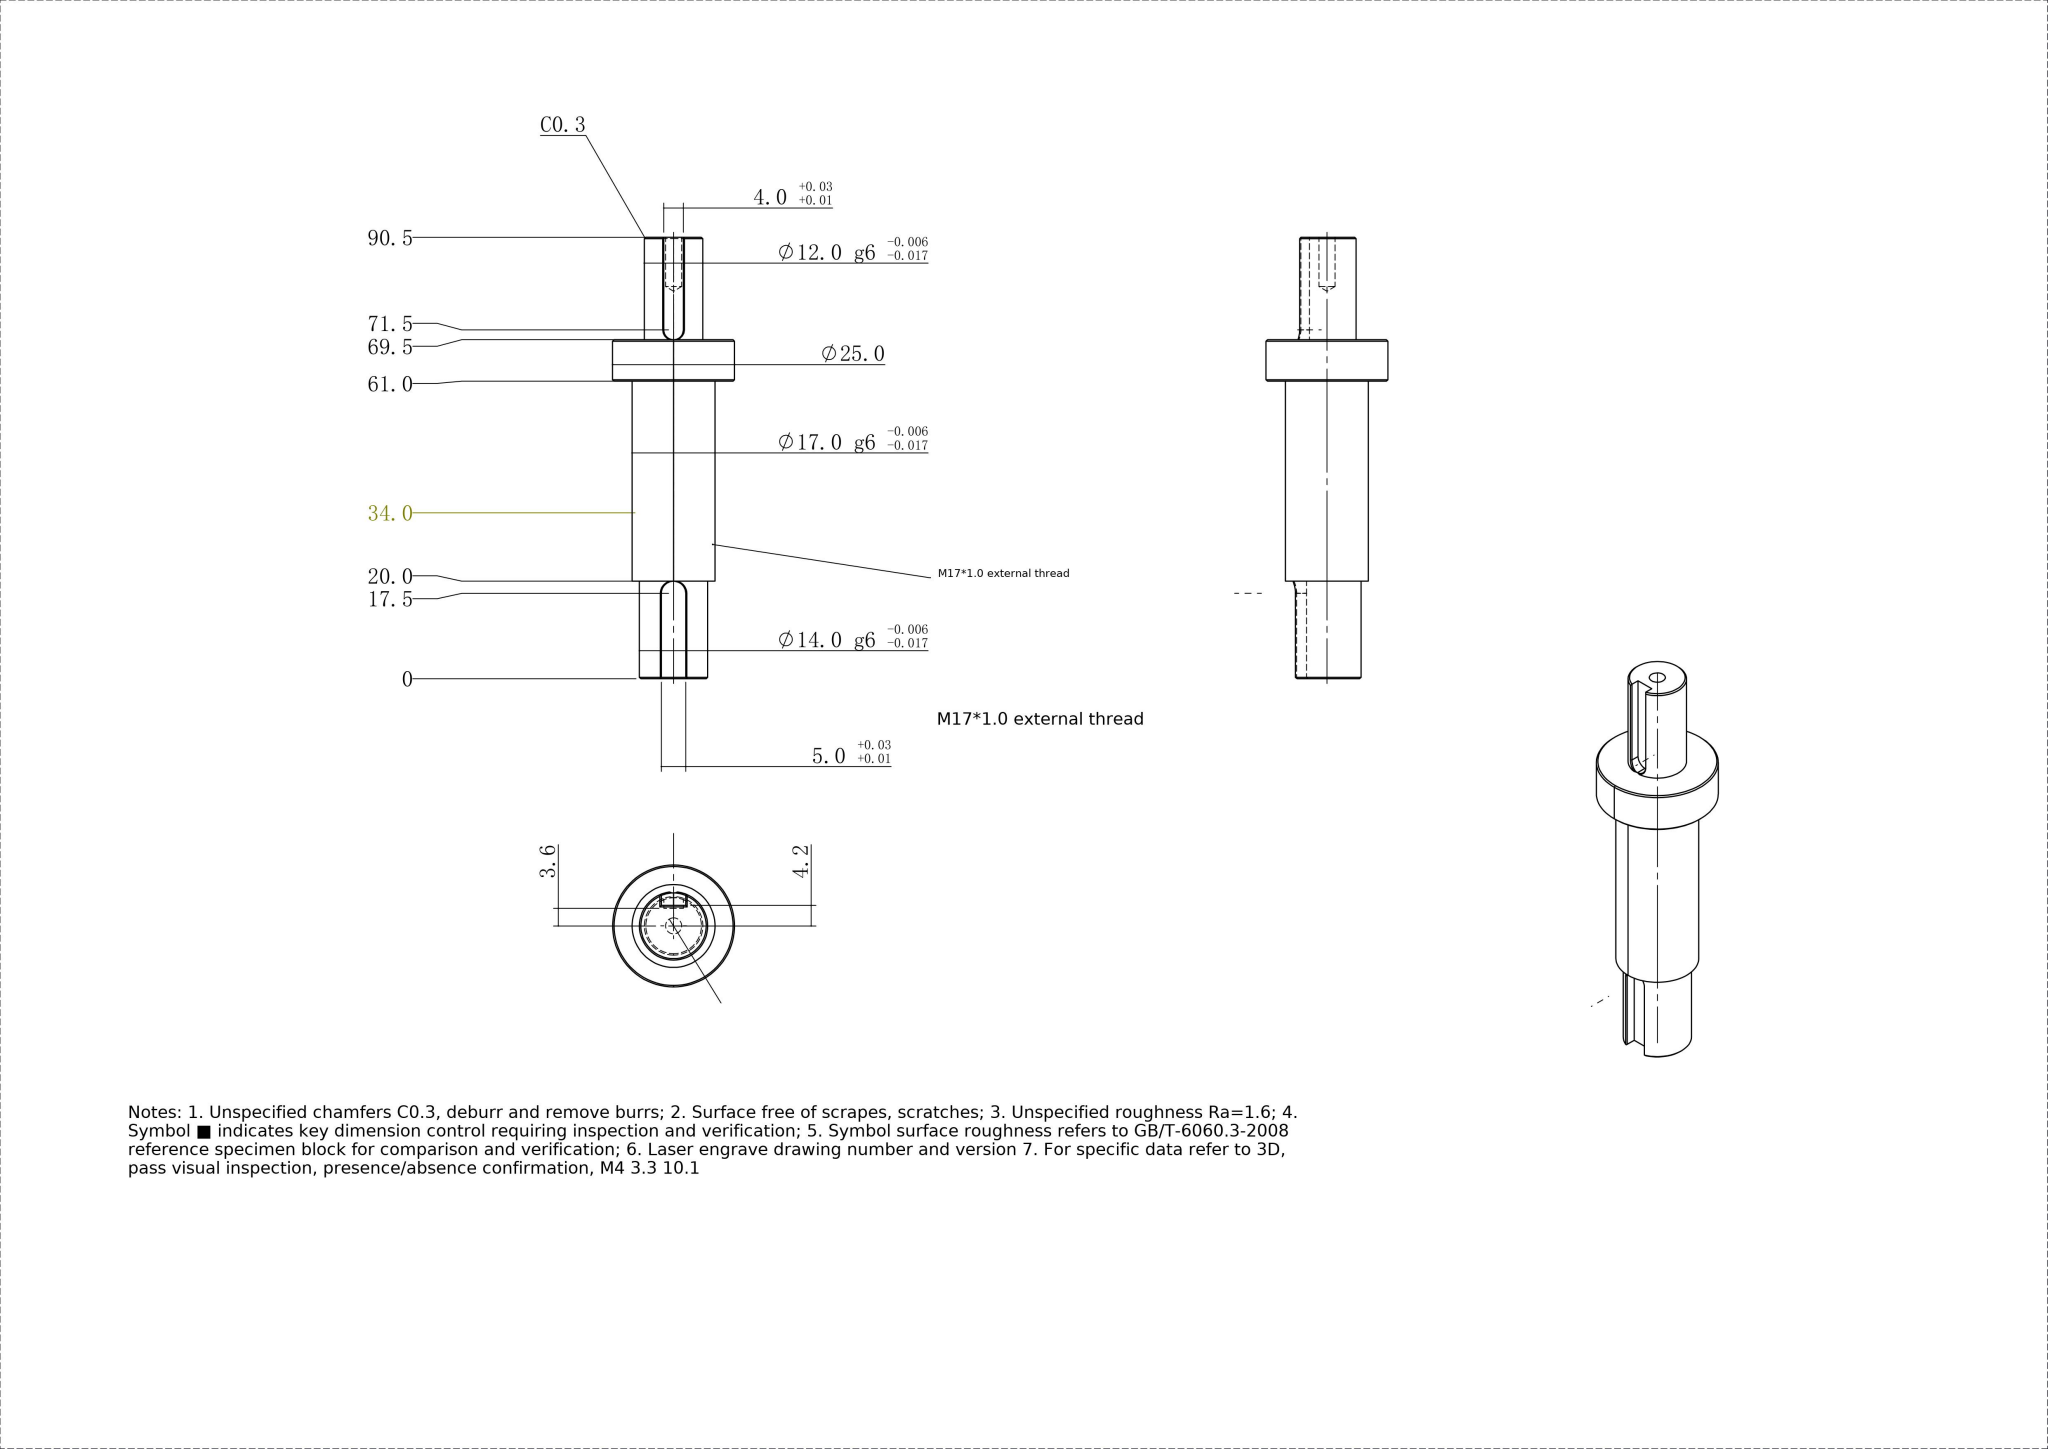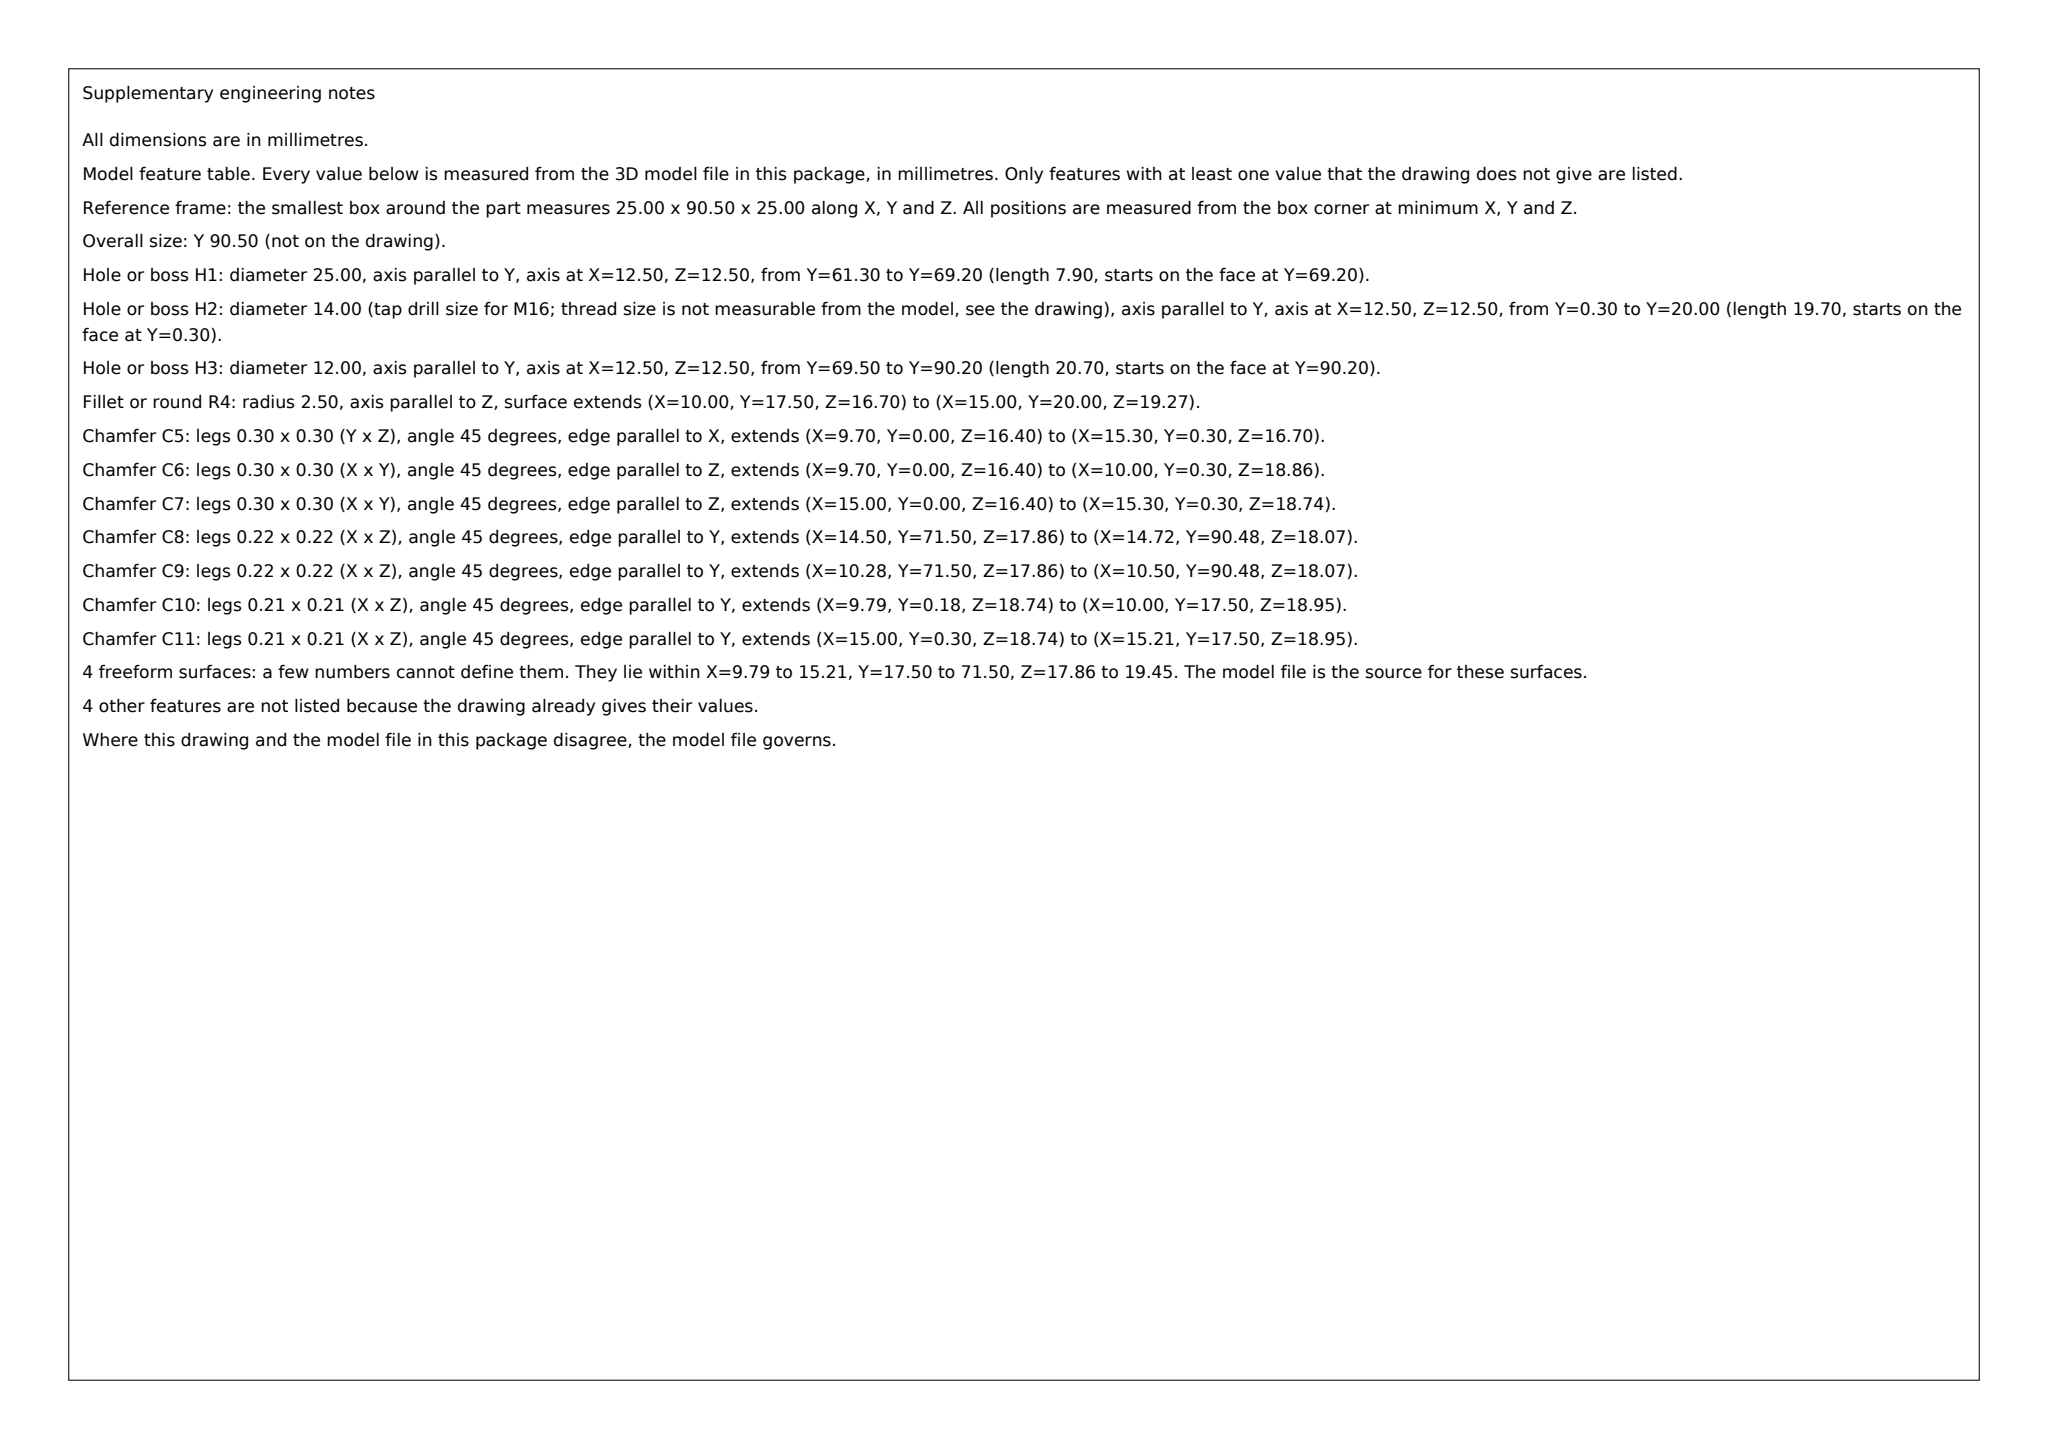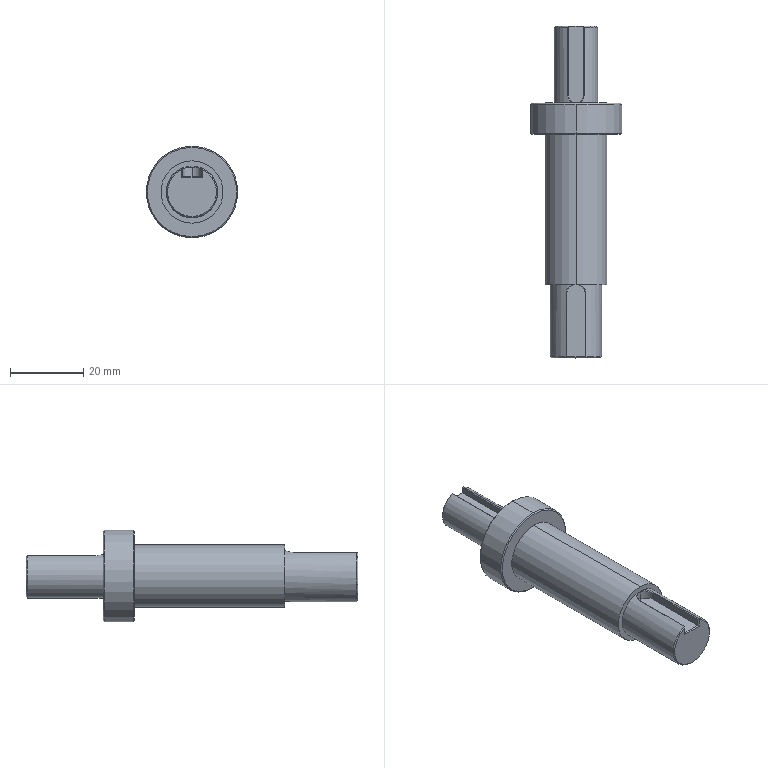Part | SolidWorks | mm | 1 solid | 45 faces | box 25 x 90.5 x 25 mm | volume 18383 mm3 | plane 19 | cylinder 13 | cone 9 | spline 4 | commonest cylinder face diameters 3.3 x2 5 x2 4 x2 17 x2 25 x2 12 x2 14 x1